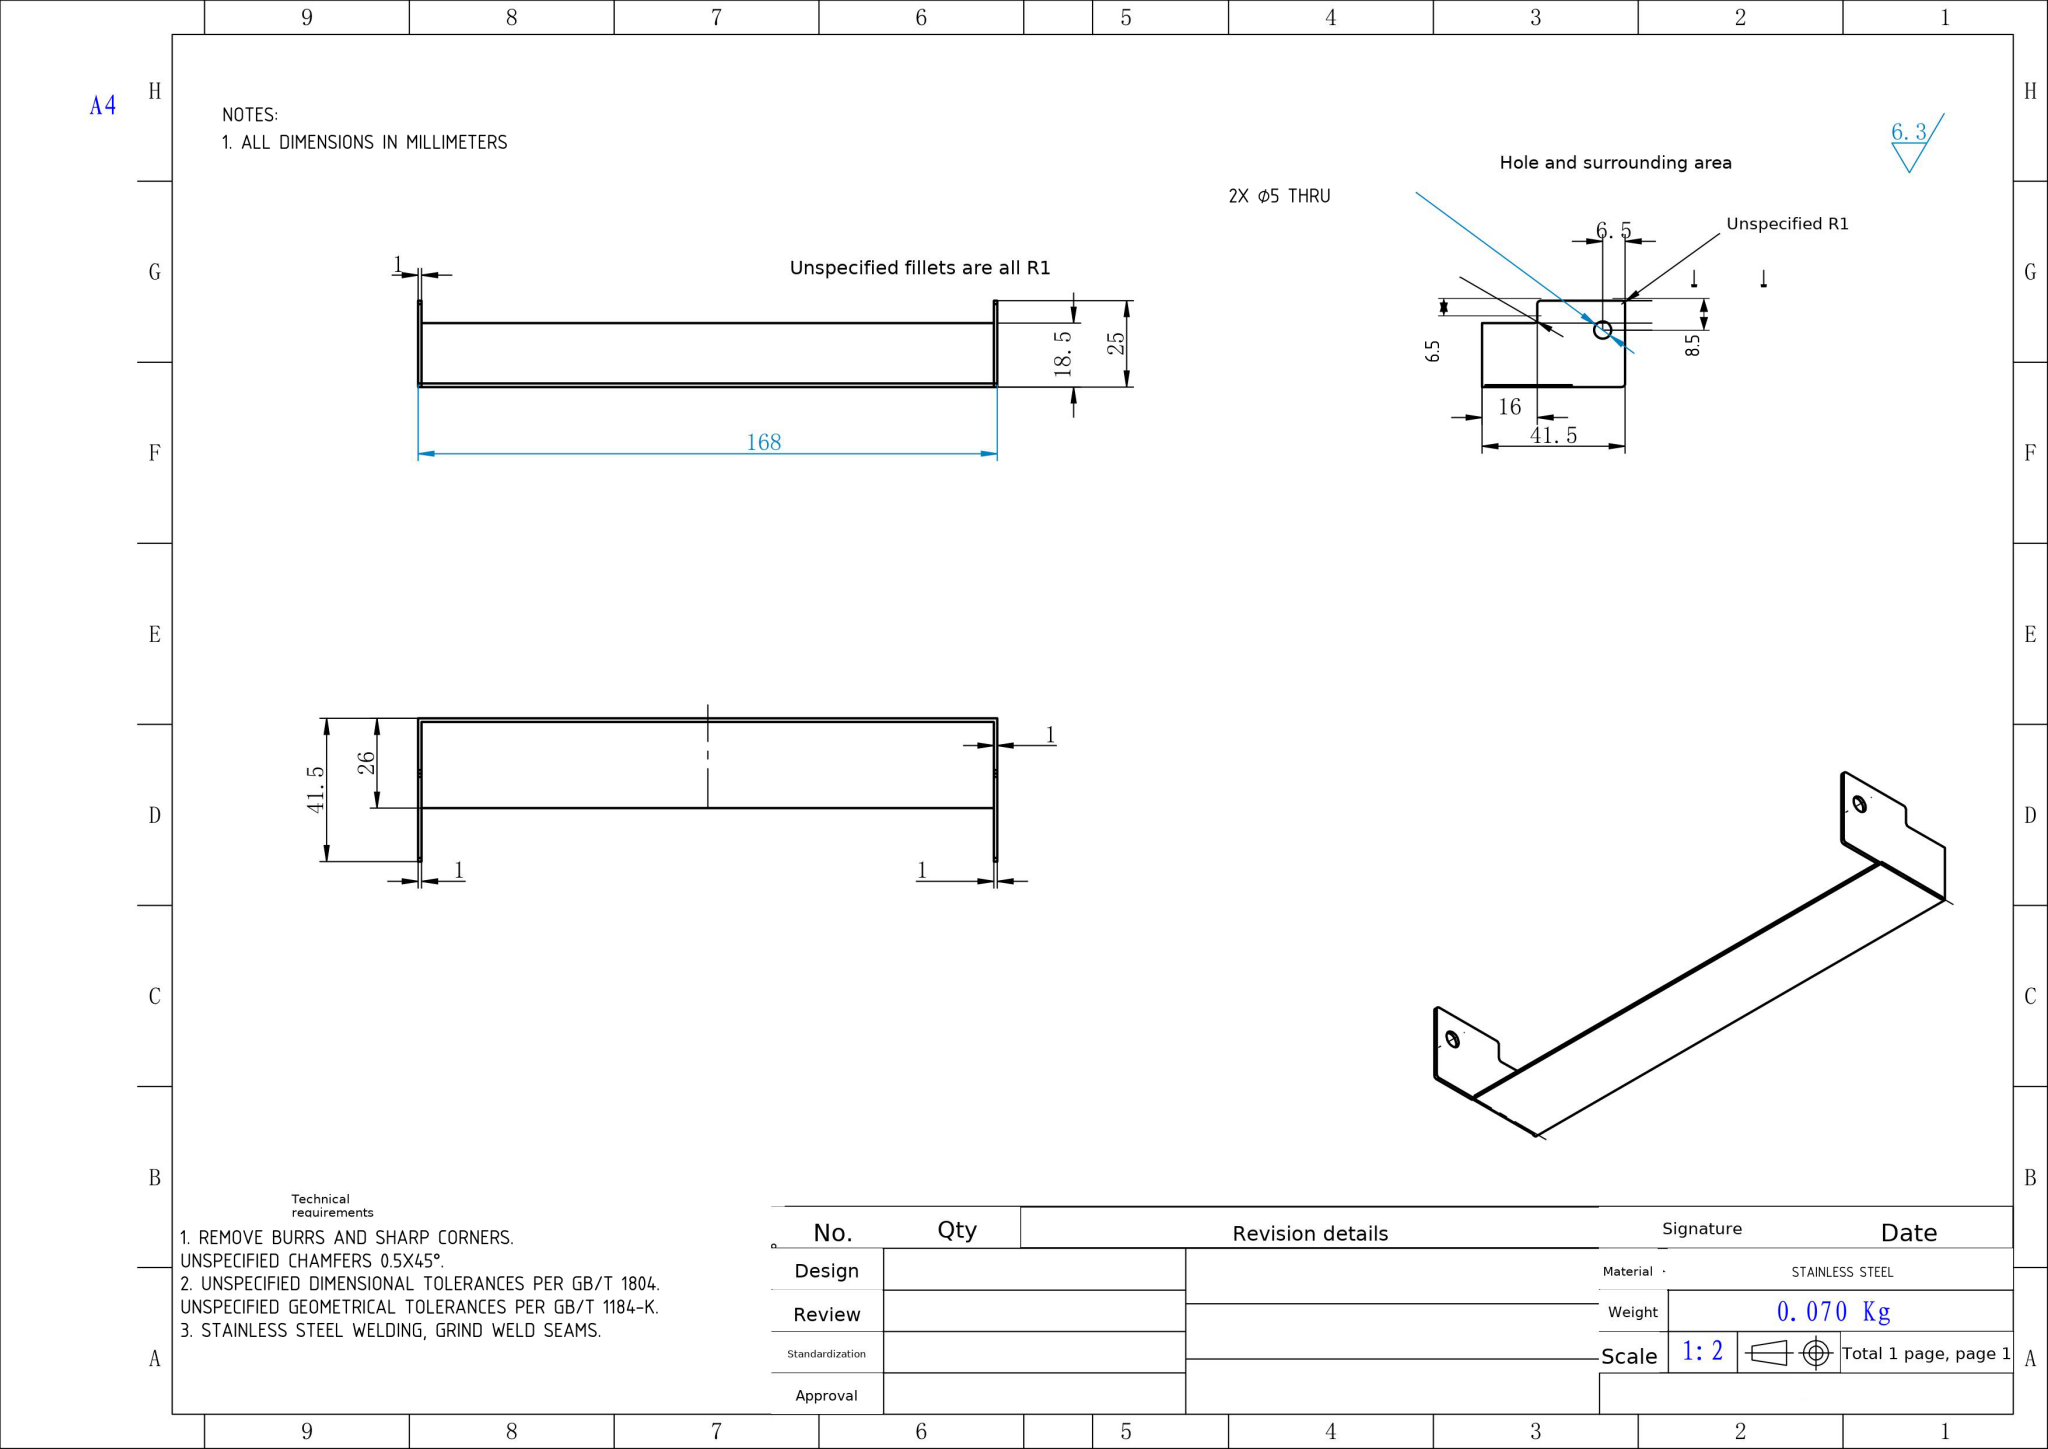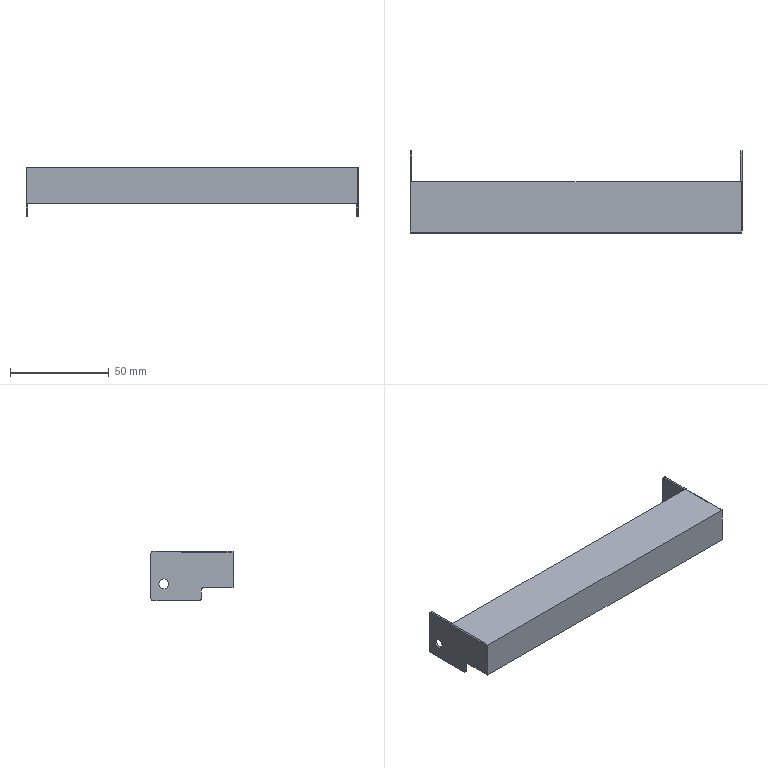Part | NX | mm | 1 solid | 34 faces | box 168 x 41.5 x 25 mm | volume 9045 mm3 | plane 20 | cylinder 14 | commonest cylinder face diameters 2 x8 5 x4 1 x2